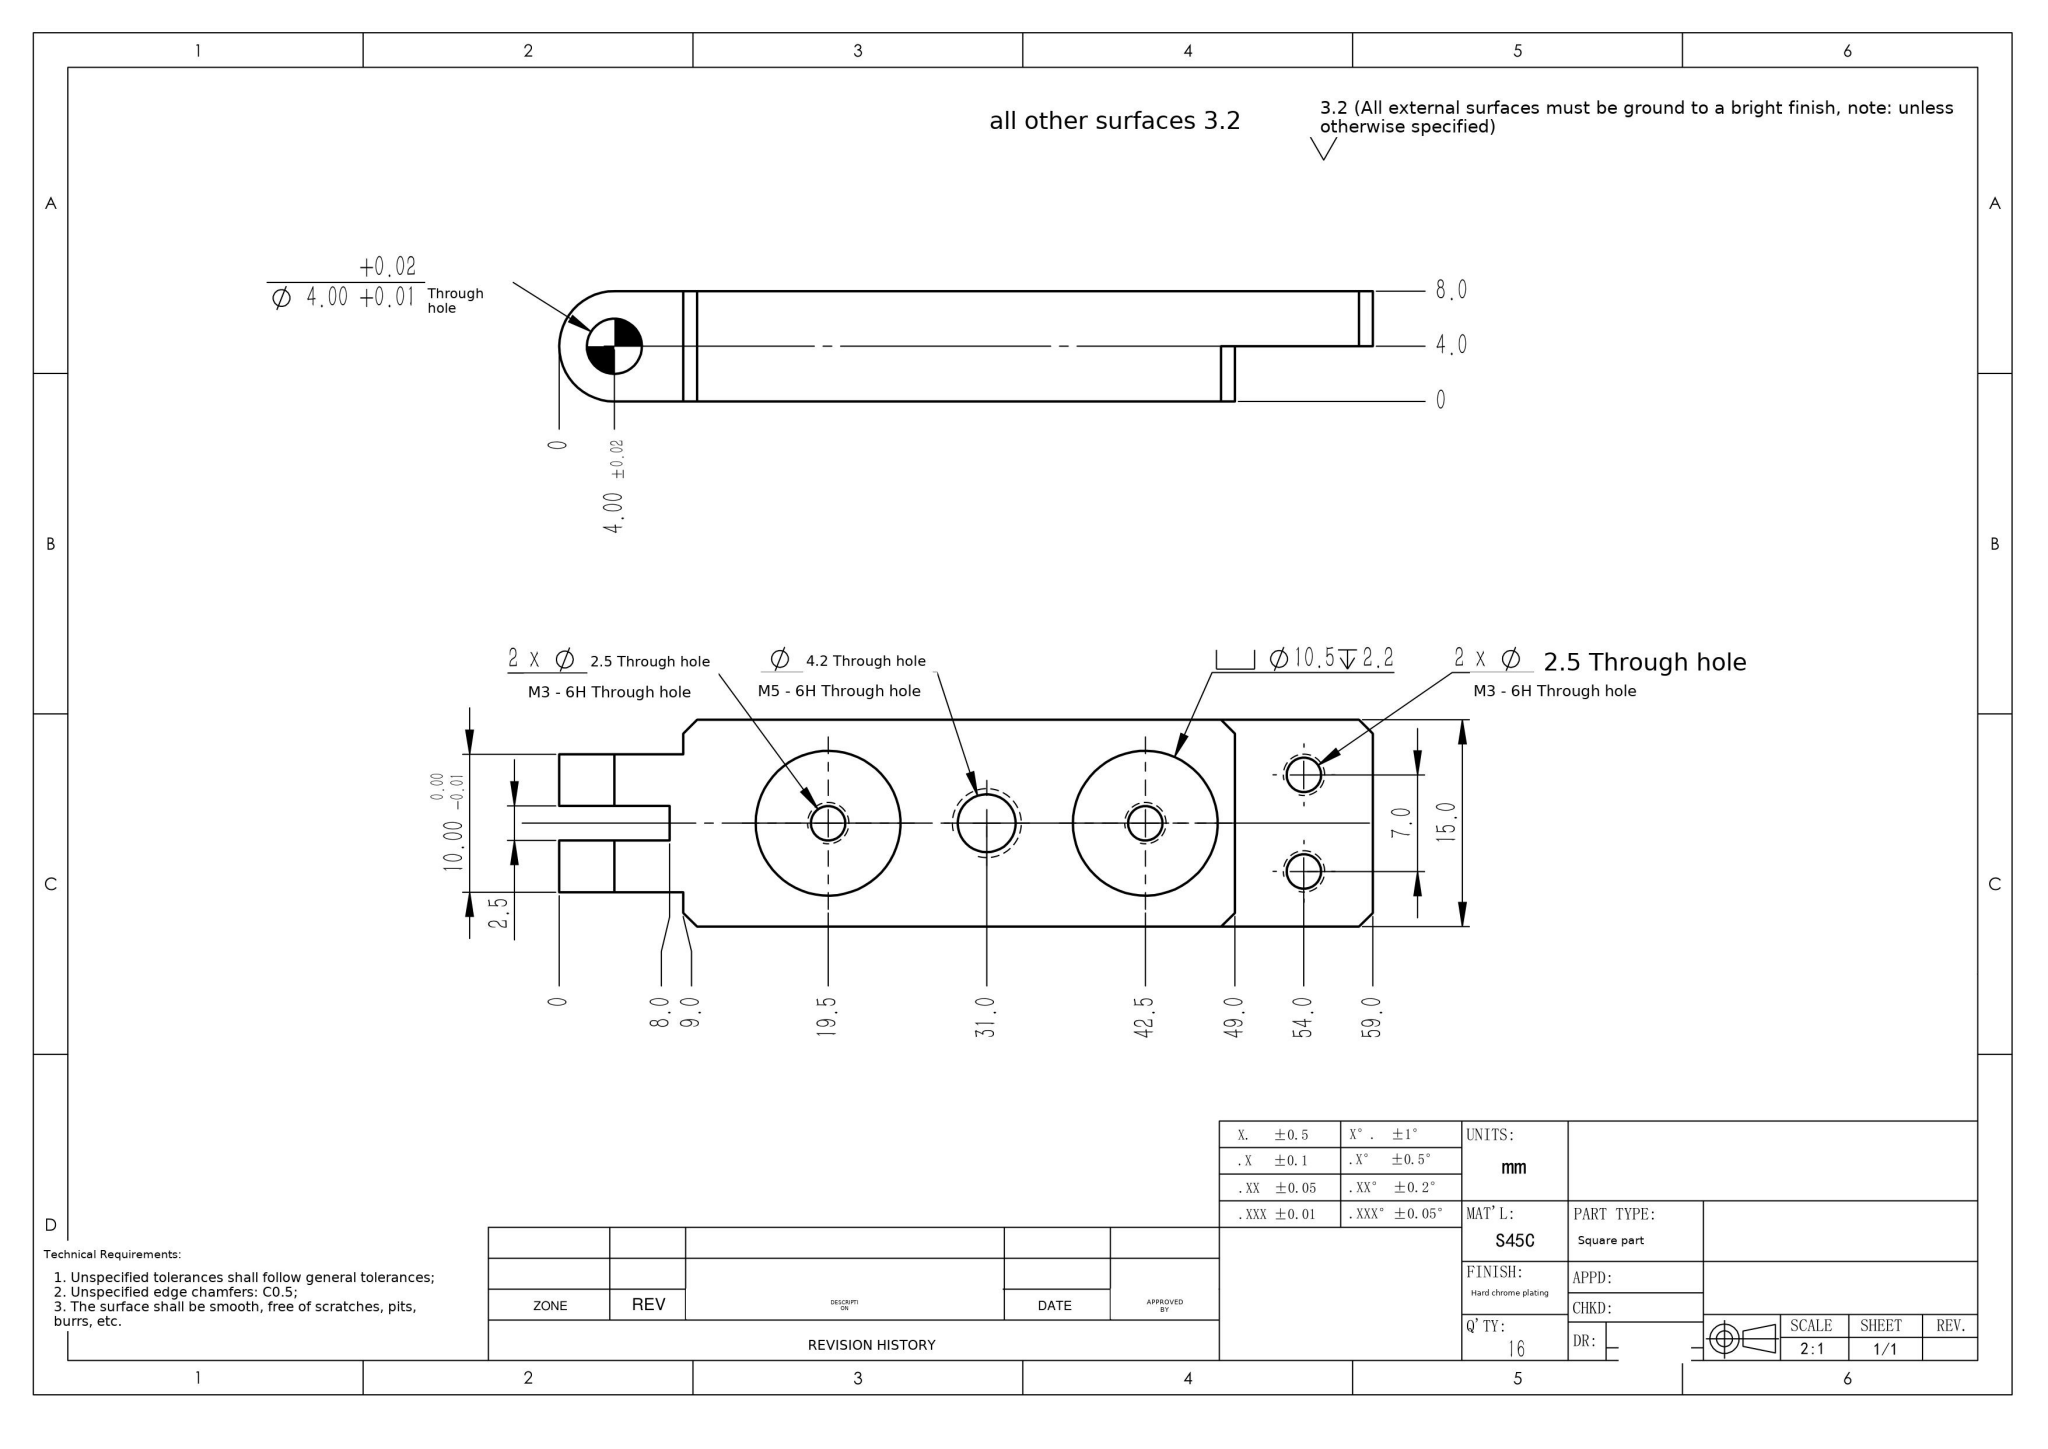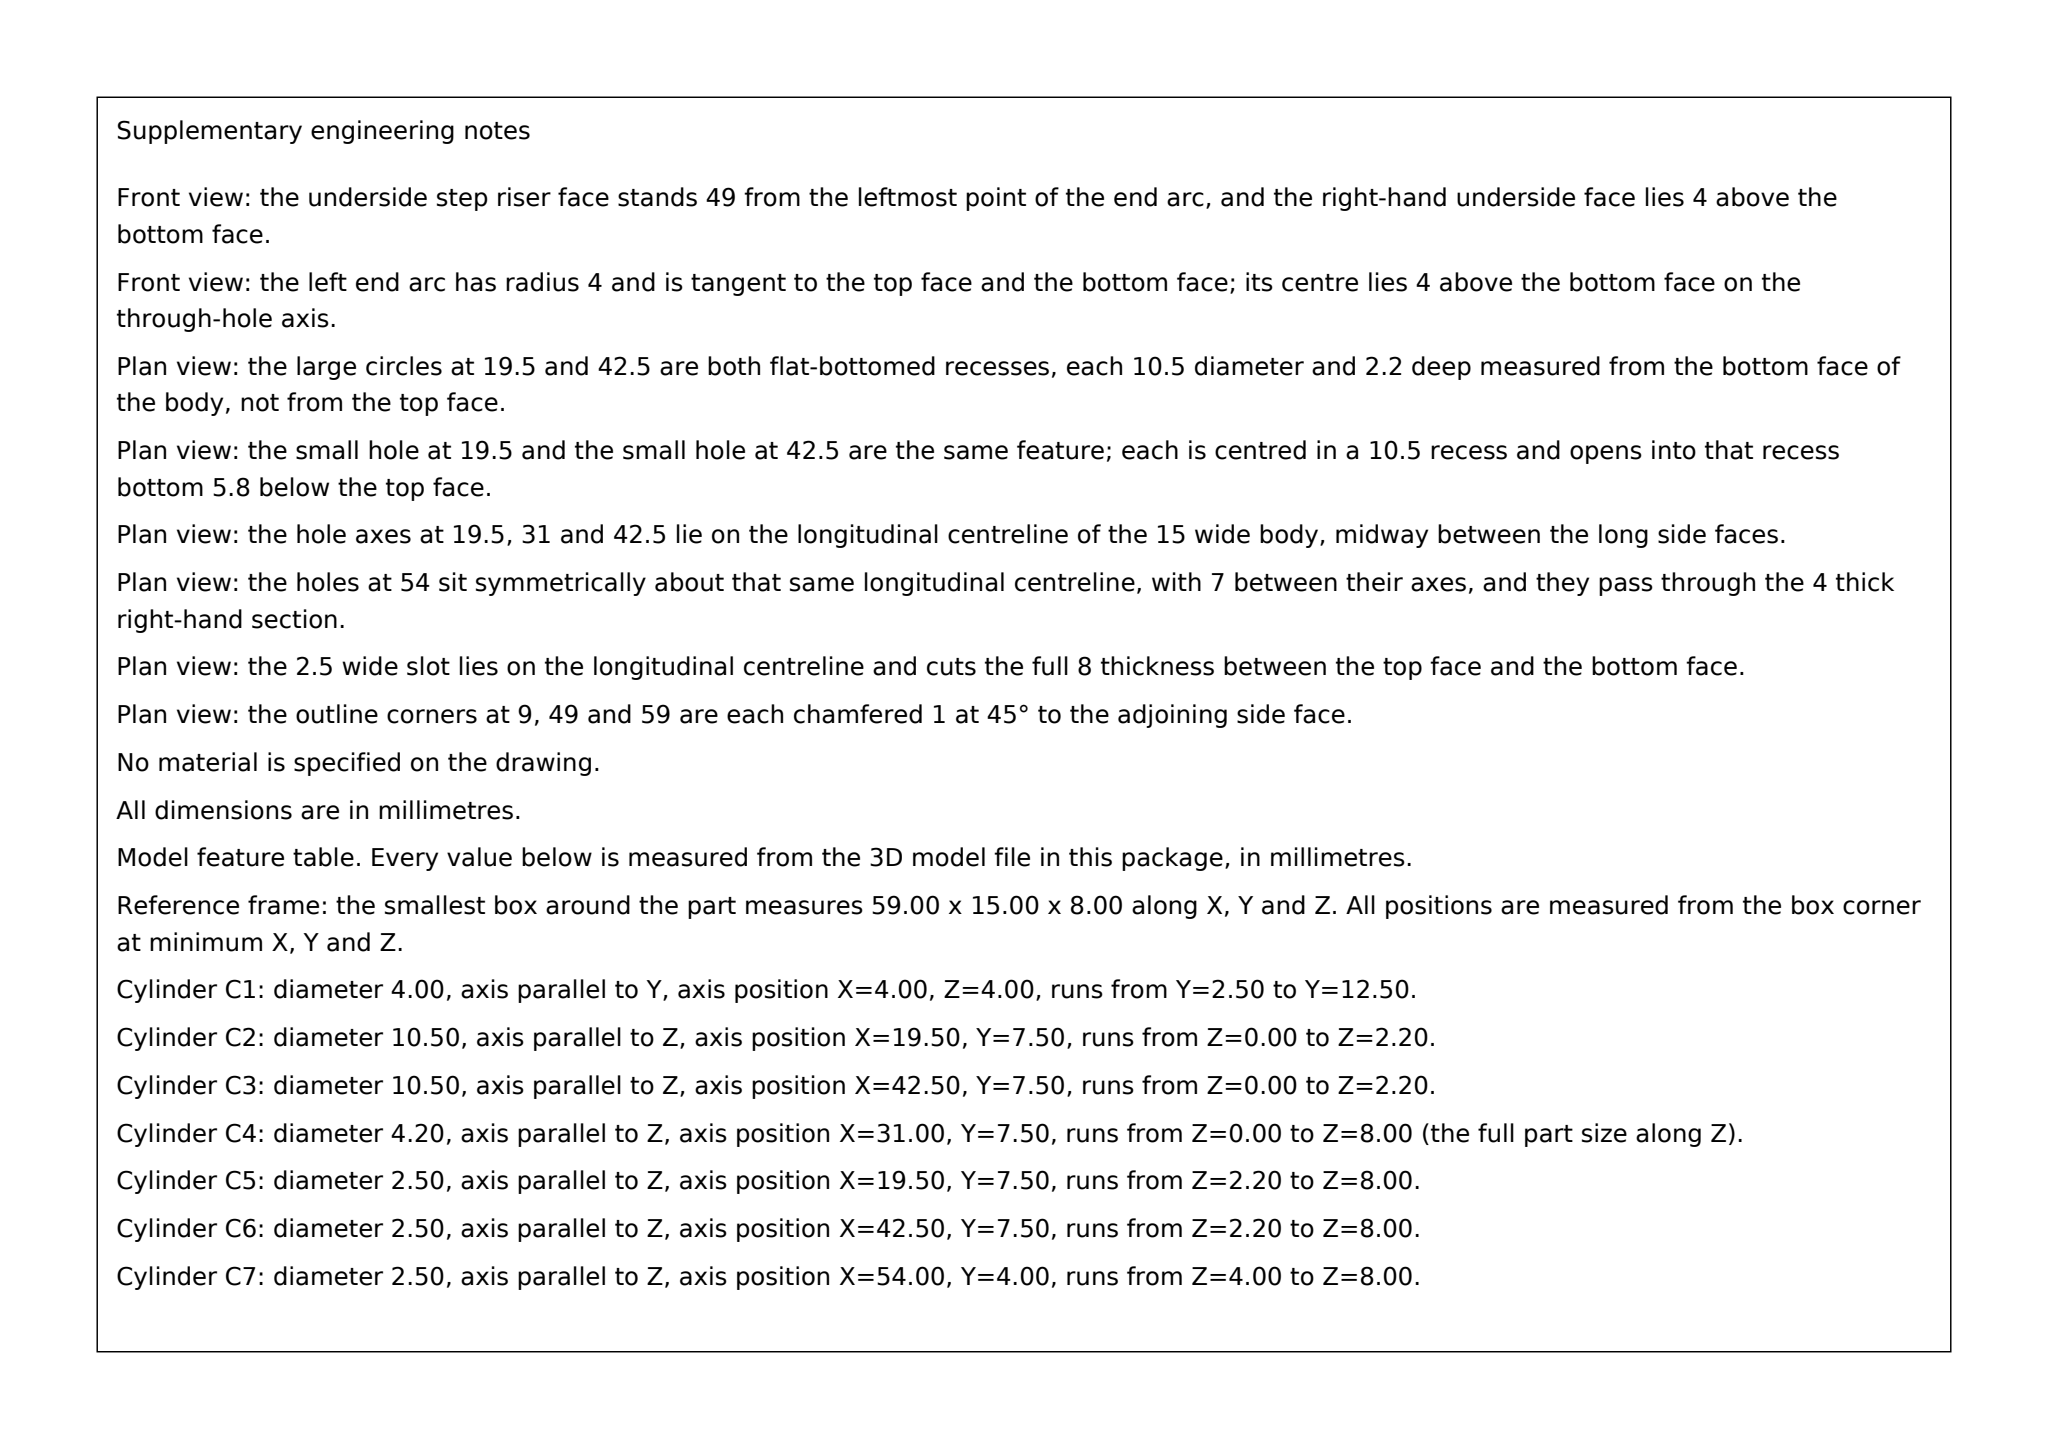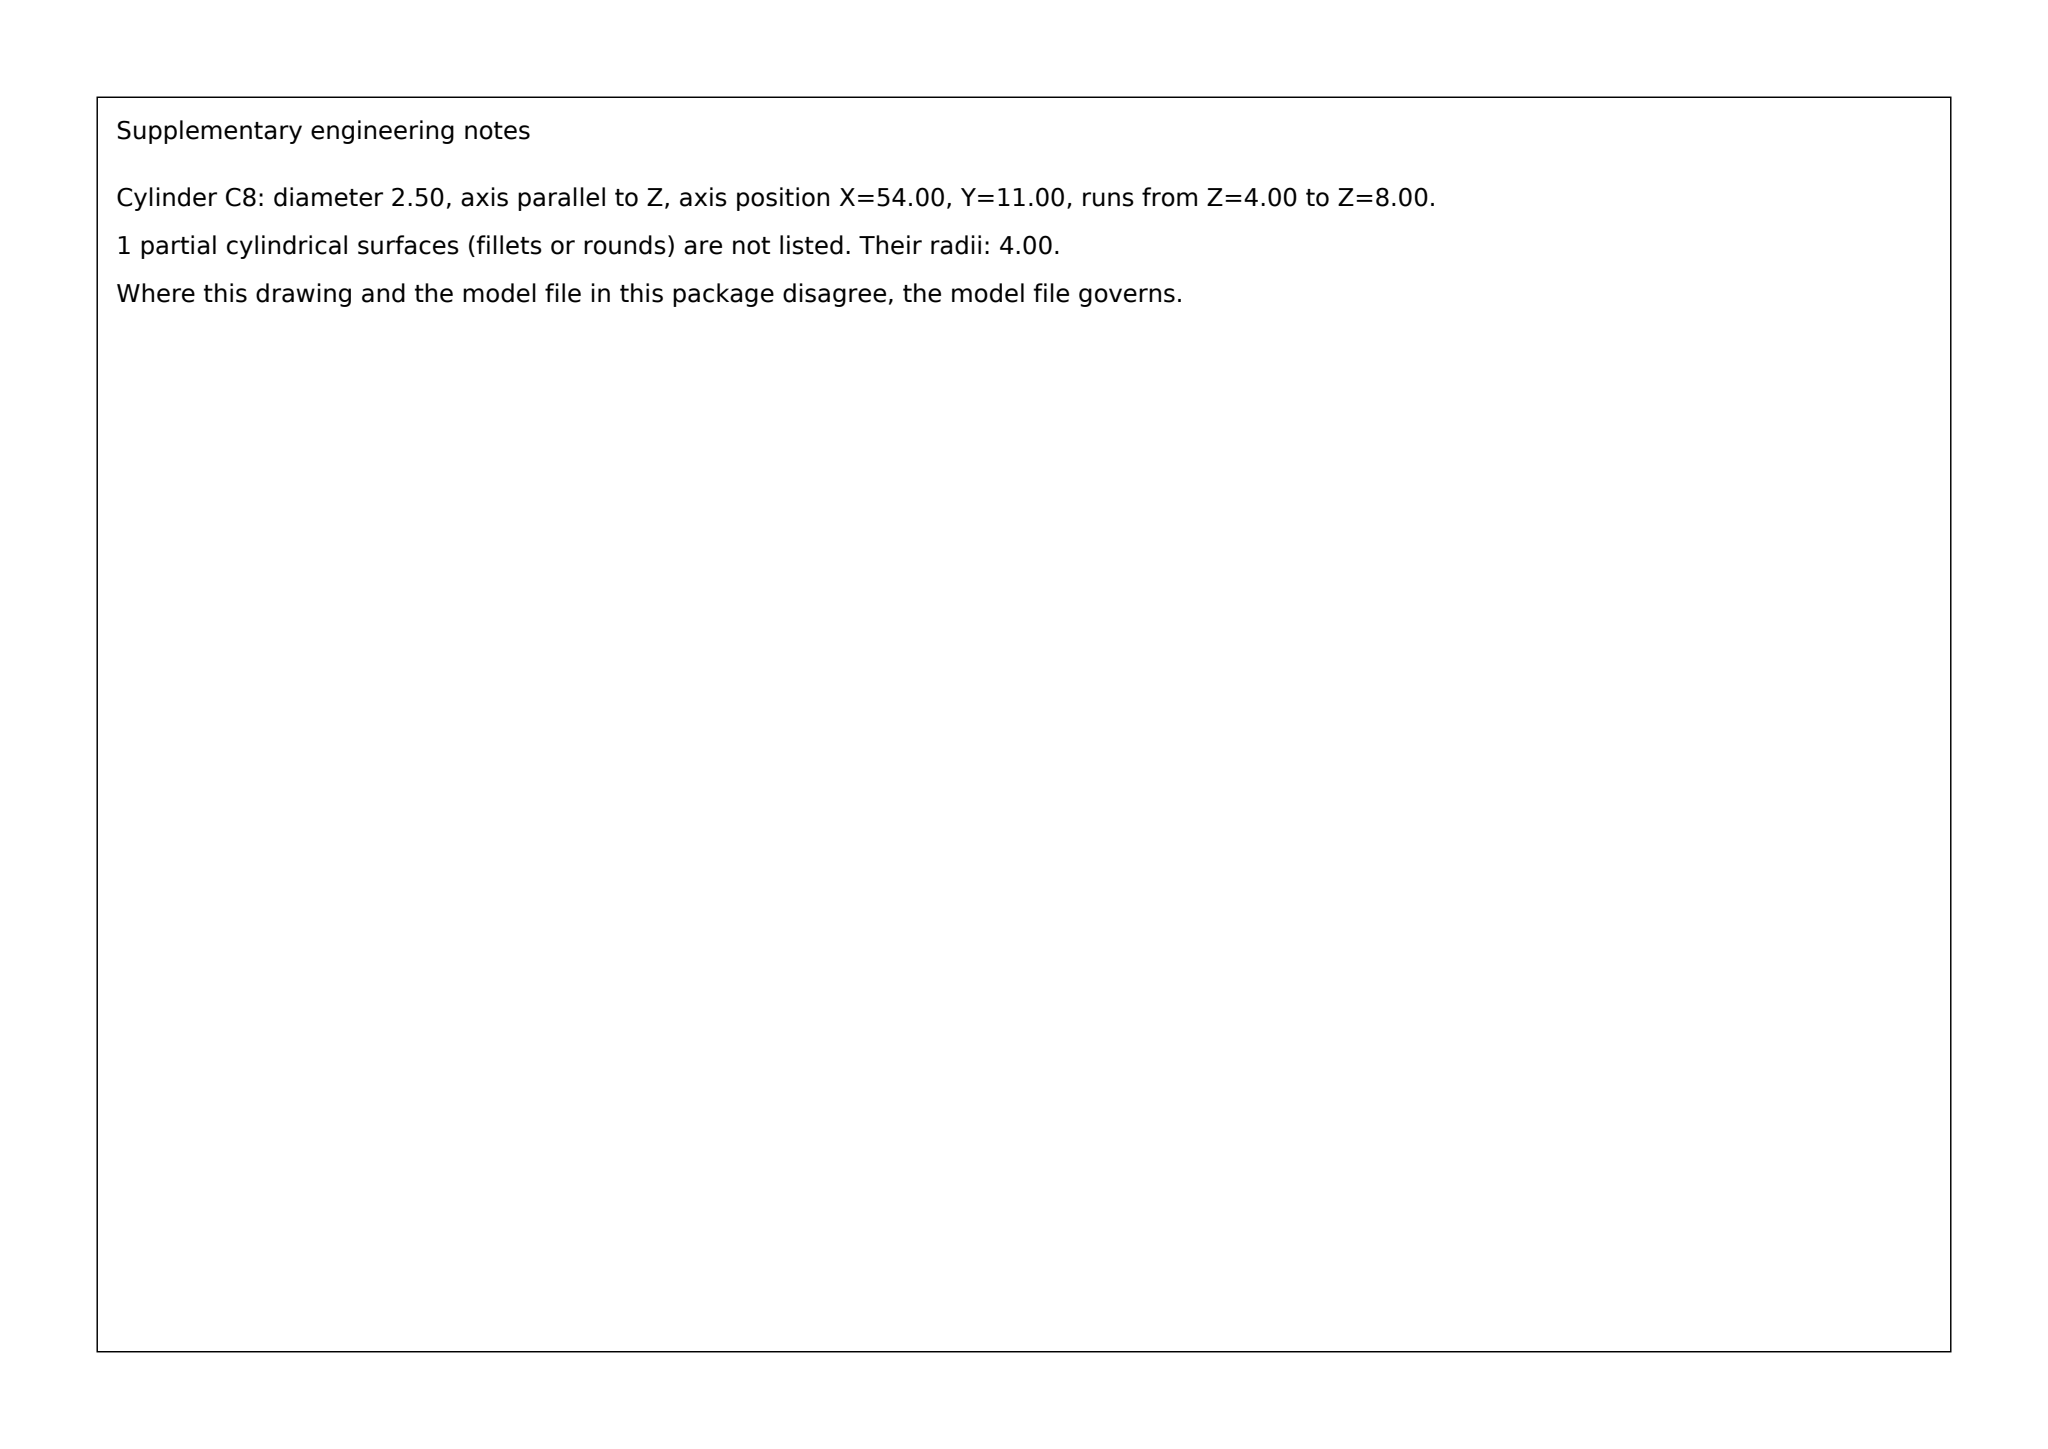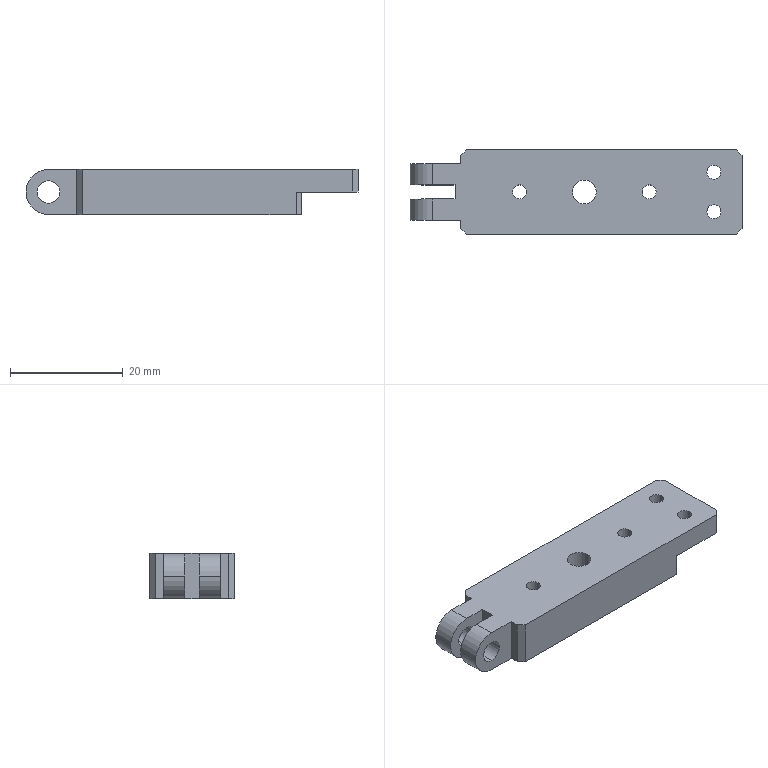Part | SolidWorks | mm | 1 solid | 44 faces | box 59 x 15 x 8 mm | volume 5210 mm3 | cylinder 22 | plane 22 | commonest cylinder face diameters 2.5 x8 10.5 x4 4 x4 8 x4 4.2 x2
Drawing notes:
FORK SLOT 2.5 WIDE x 8.0 DEEP; PRONG THK 3.75 EA SIDE | from the solid: y-planes 6.25/8.75 give 2.5 gap; y 2.5-6.25 & 8.75-12.5 = 3.75 prongs; slot end plane x=8.0
FORK-TO-BODY STEP AT 9.0: 2.5 PER SIDE, 10.0 TO 15.0 WIDE | from the solid: x-planes at 9.0 (count 2); y 2.5 & 12.5 fork faces vs y 0 & 15.0 body faces
2X Ø10.5 DP 2.2 FROM 0 FACE (BOTTOM) IN SIDE VIEW | from the solid: Ø10.5 cyls at x19.5 & x42.5, y7.5, L2.2; z-planes at 2.2 (count 2) above z=0 face
FORK END R4.0 (Ø8.0), C/L 4.00 FROM END & 4.00 FROM 0 FACE | from the solid: Ø8.0 y-axis cyls at x=4.0, z=4.0, L3.75 (x2 prongs), coaxial with Ø4.00 hole
TOP VIEW: 2X CHAM 2.5 X 45 DEG AT 49.0 BODY-TO-TAB CORNERS | from the solid: x-plane at 49.0 (step/tab face) with side faces y=0 and y=15.0 reduced to y=2.5 / y=12.5 planes; equal 2.5 legs => 2.5 x 45 deg chamfer each side
SIDE VIEW: BODY-TO-TAB THICKNESS STEP LOCATED AT 49.0 FROM 0 END (FORK END); BODY THK 8.0, TAB THK 4.0 MEASURED FROM 0 FACE (BOTTOM) | from the solid: axis_planes [x,49.0] step face; axis_planes [z,4.0] and [z,8.0] with bbox_xyz z=8.0